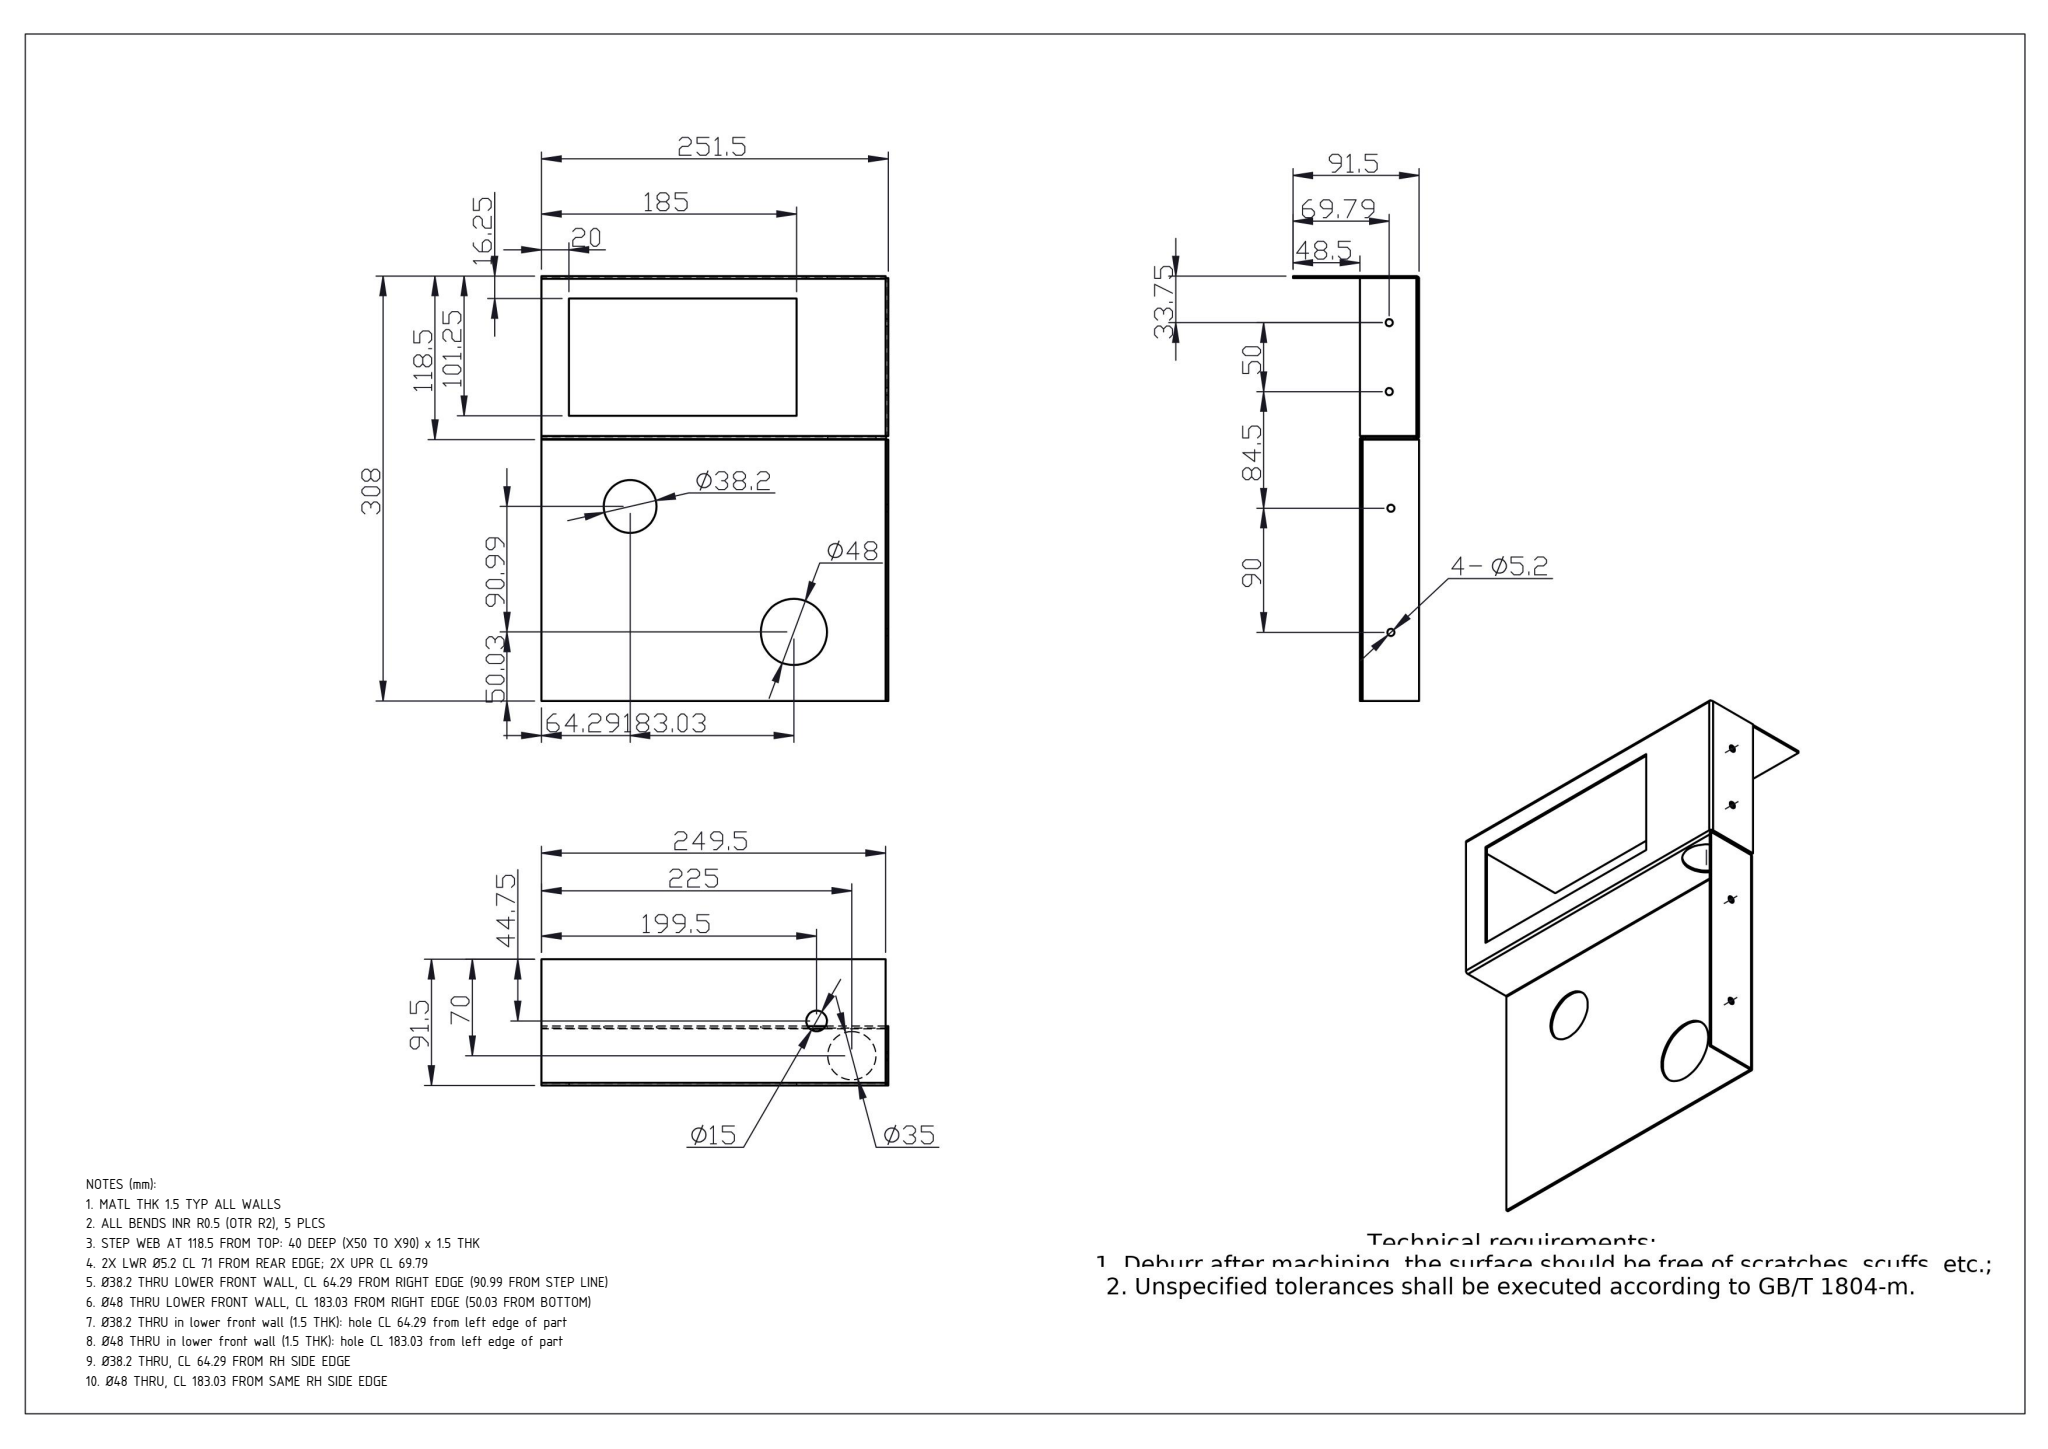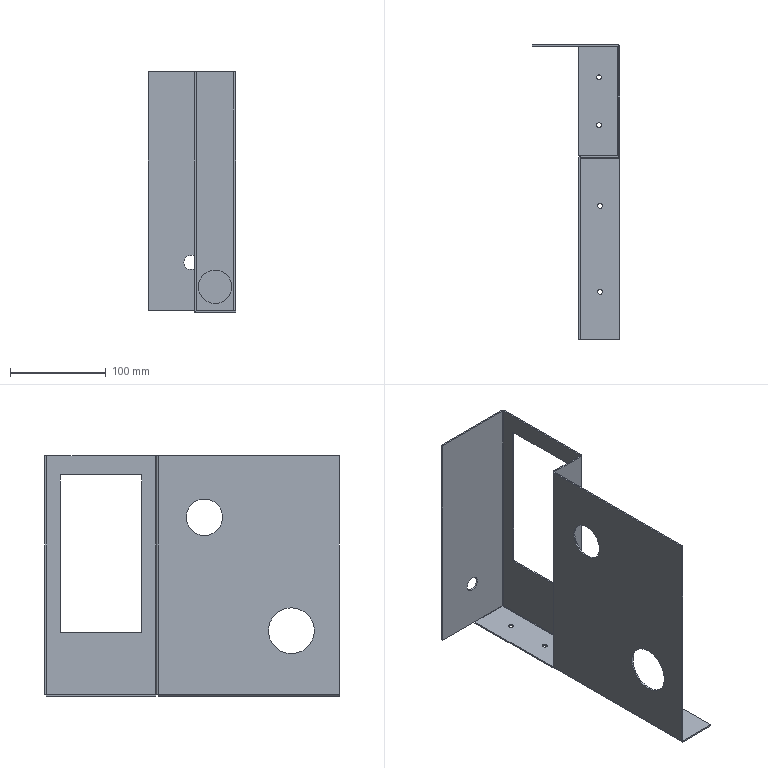Part | SolidWorks | mm | 1 solid | 69 faces | box 91.5 x 308 x 251.5 mm | volume 156197 mm3 | plane 43 | cylinder 26 | commonest cylinder face diameters 5.2 x8 4 x5 1 x5 38.204 x2 48.004 x2 15 x2 35 x2
Drawing notes:
MATL THK 1.5 TYP ALL WALLS | from the solid: Face pairs 48.5/50, 90/91.5, 0/1.5, 306.5/308; all hole cyl length 1.5
ALL BENDS INR R0.5 (OTR R2), 5 PLCS | from the solid: Ø1.0 inner / Ø4.0 outer cyls on 5 bend lines: y-axis x50.5 & x89.5 at z2.0; z-axis x50.5/y189.5, x89.5/y192.0, x89.5/y306.0
STEP WEB AT 118.5 FROM TOP: 40 DEEP (X50 TO X90) x 1.5 THK | from the solid: y planes 189.5/190/191.5/192 (308-189.5=118.5); x faces 50 and 90, web thk 1.5
2X LWR Ø5.2 CL 71 FROM REAR EDGE; 2X UPR CL 69.79 | from the solid: Ø5.2 axis z at x=71.0 (y=49.75,139.75) and x=69.79 (y=224.25,274.25)
Ø38.2 THRU LOWER FRONT WALL, CL 64.29 FROM RIGHT EDGE (90.99 FROM STEP LINE) | from the solid: cylinders: [38.204,"x",[null,141.02,187.21],1.5] -> 251.5-187.21=64.29 from z-max edge
Ø48 THRU LOWER FRONT WALL, CL 183.03 FROM RIGHT EDGE (50.03 FROM BOTTOM) | from the solid: cylinders: [48.004,"x",[null,50.03,68.47],1.5] -> 251.5-68.47=183.03 from z-max edge; y=50.03 from bottom
Ø38.2 THRU in lower front wall (1.5 THK): hole CL 64.29 from left edge of part | from the solid: cylinder dia 38.204, axis x, pos [y=141.02, z=187.21], length 1.5; bbox z=251.5 so 251.5-187.21=64.29
Ø48 THRU in lower front wall (1.5 THK): hole CL 183.03 from left edge of part | from the solid: cylinder dia 48.004, axis x, pos [y=50.03, z=68.47], length 1.5; bbox z=251.5 so 251.5-68.47=183.03
Ø38.2 THRU, CL 64.29 FROM RH SIDE EDGE | from the solid: cylinder dia 38.204, axis x, pos z=187.21; bbox z=251.5 (251.5-187.21=64.29)
Ø48 THRU, CL 183.03 FROM SAME RH SIDE EDGE | from the solid: cylinder dia 48.004, axis x, pos z=68.47; bbox z=251.5 (251.5-68.47=183.03)